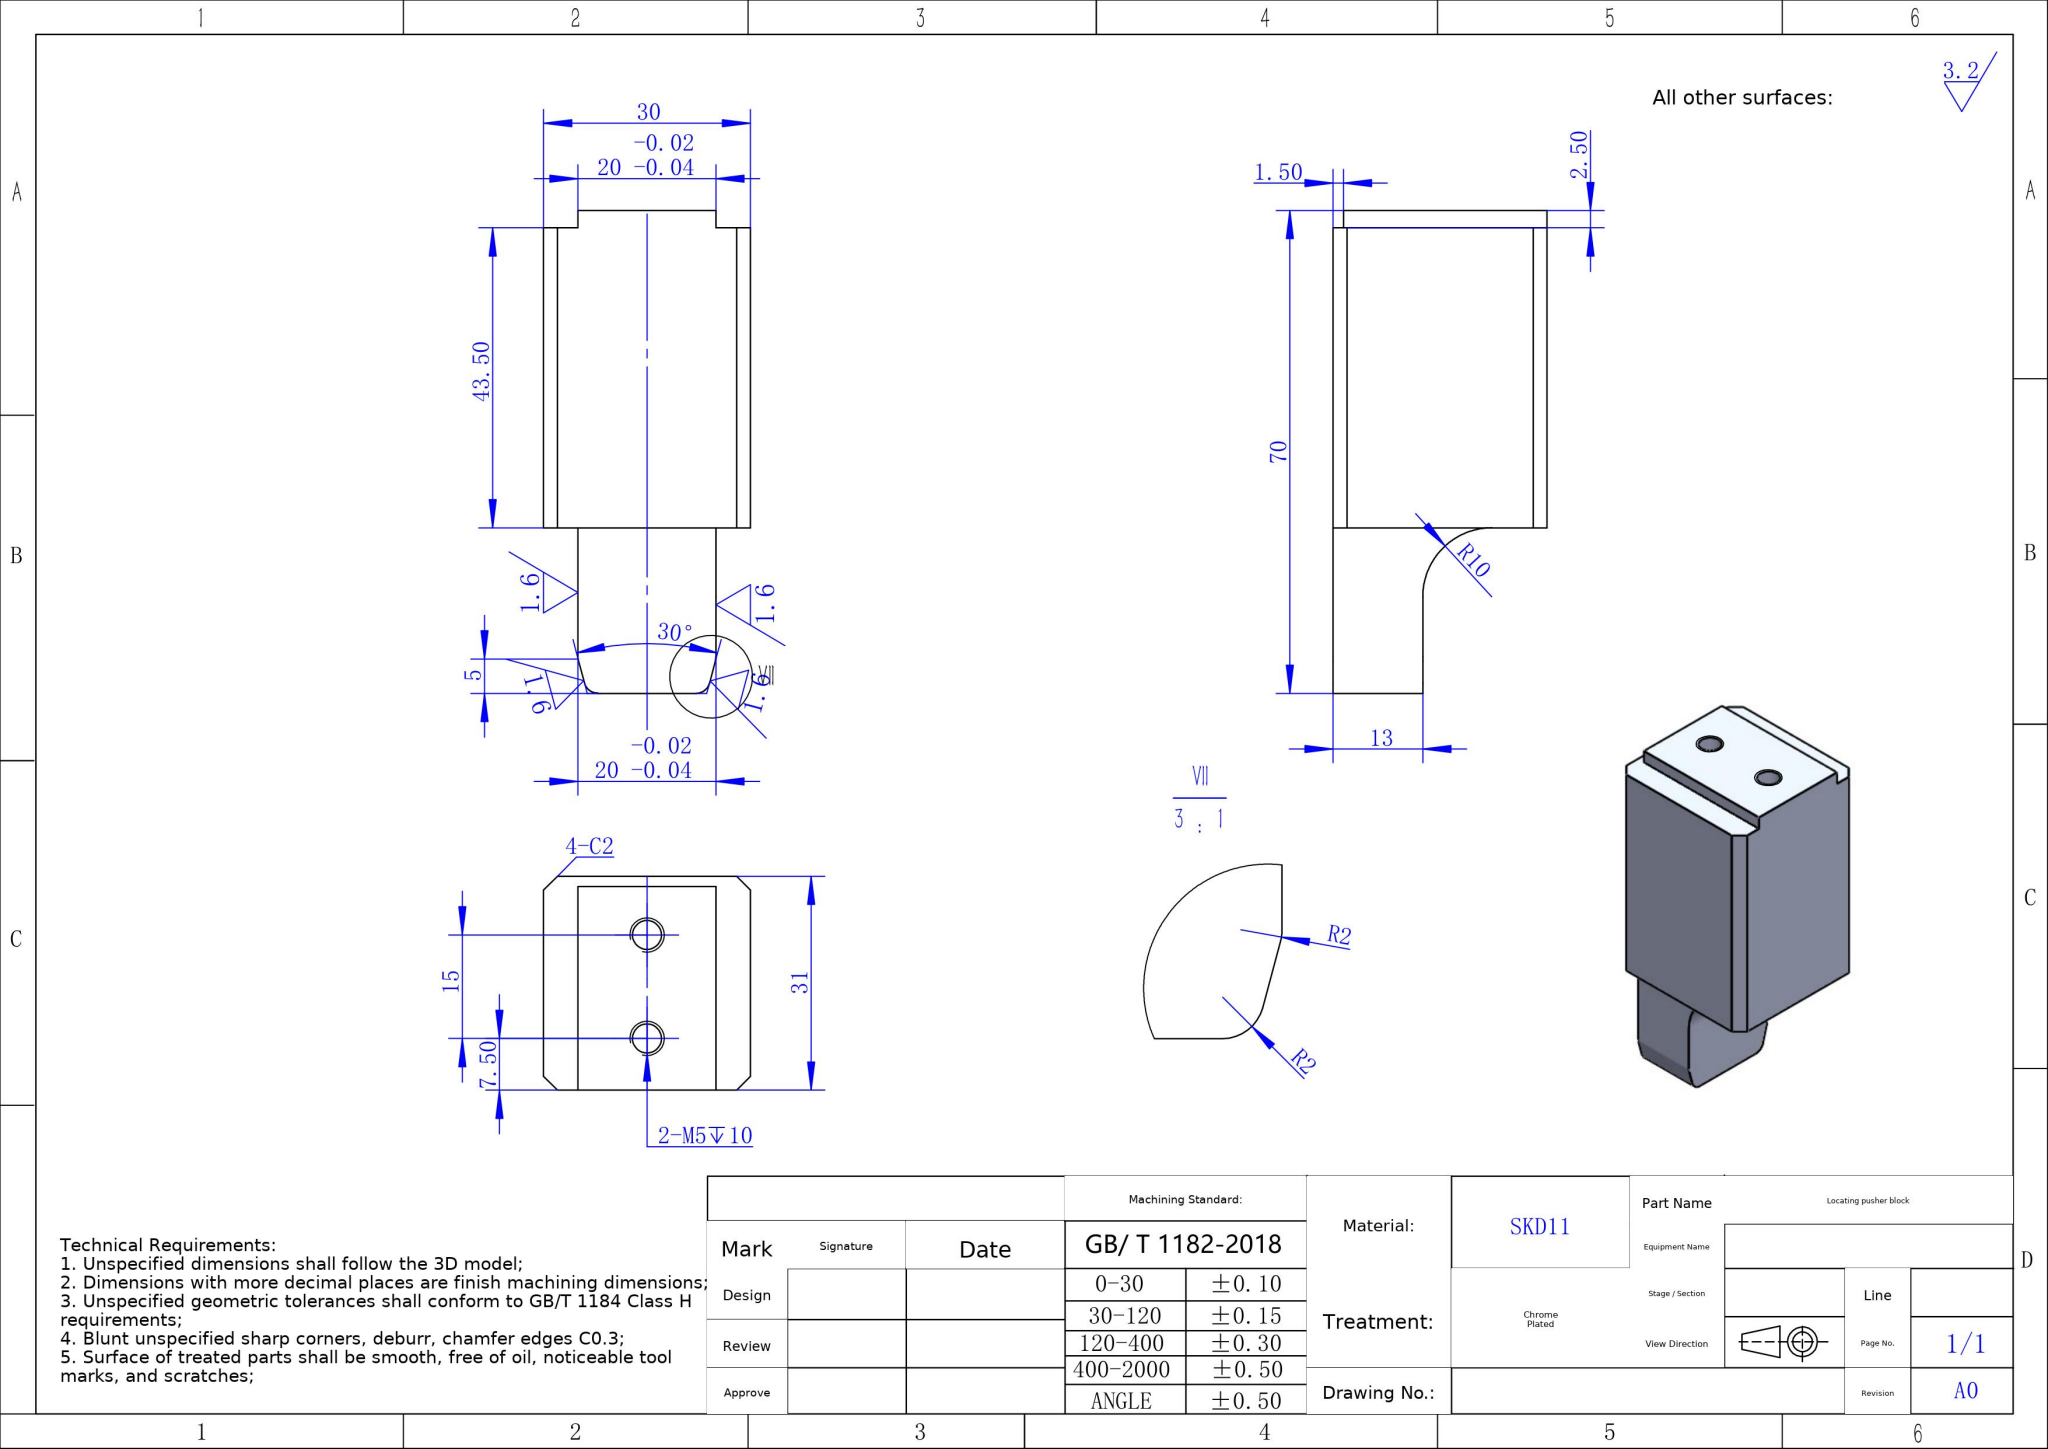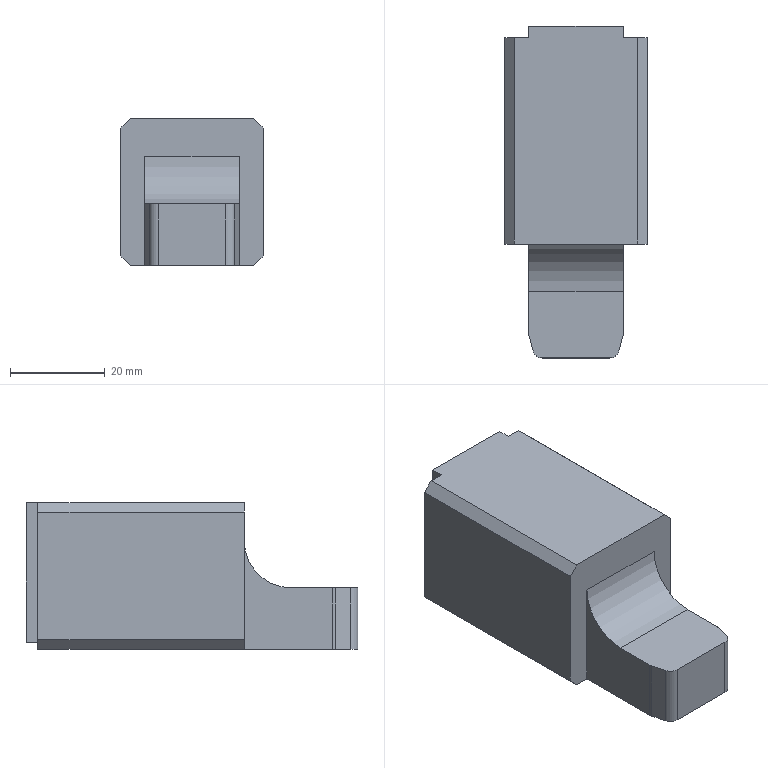Part | SolidWorks | mm | material SKD11 | 1 solid | 33 faces | box 30 x 70 x 31 mm | volume 47753 mm3 | plane 20 | cylinder 9 | cone 4 | commonest cylinder face diameters 4.2 x4 4 x4 20 x1
build123d program:
from build123d import *

# Parameters (mm, degrees)
SKETCH1_W             = 30
SKETCH1_H             = 43.5
BOSS_EXTRUDE1_DEPTH   = 31
CHAMFER1_SIZE         = 2
SKETCH2_W             = 20
SKETCH2_H             = 2.5
BOSS_EXTRUDE2_DEPTH   = 29.5
M5_TAPPED_HOLE1_D     = 4.2
M5_TAPPED_HOLE1_DEPTH = 14
M5_TAPPED_HOLE1_TIP   = 1.262
SKETCH5_W             = 13
SKETCH5_H             = 24
BOSS_EXTRUDE3_DEPTH   = 10
FILLET1_R             = 10
CUT_EXTRUDE1_DEPTH    = 20
FILLET2_R             = 2


with BuildPart() as part:
    # Sketch1 → Boss-Extrude1 (new body)
    with BuildSketch(Plane.XY):
        Rectangle(SKETCH1_W, SKETCH1_H)
    extrude(amount=BOSS_EXTRUDE1_DEPTH)

    # Chamfer1
    chamfer1_edges = [part.edges().sort_by_distance(p)[0] for p in [
        (-15, 0, 31),
        (15, 0, 31),
        (-15, 0, 0),
        (15, 0, 0),
    ]]
    chamfer(chamfer1_edges, length=CHAMFER1_SIZE)

    # Sketch2 → Boss-Extrude2 (add)
    with BuildSketch(Plane.XY.offset(31)):
        with Locations((0, 23)):
            Rectangle(SKETCH2_W, SKETCH2_H)
    extrude(amount=-BOSS_EXTRUDE2_DEPTH)

    # M5 Tapped Hole1
    with Locations(Plane(origin=(0, 24.25, 0), x_dir=(1, 0, 0), z_dir=(0, 1, 0))):
        with Locations((0, -23.5), (0, -8.5)):
            Hole(M5_TAPPED_HOLE1_D / 2, depth=M5_TAPPED_HOLE1_DEPTH)
            with Locations((0, 0, -(M5_TAPPED_HOLE1_DEPTH + M5_TAPPED_HOLE1_TIP / 2))):  # 118° drill point
                Cone(0, M5_TAPPED_HOLE1_D / 2, M5_TAPPED_HOLE1_TIP, mode=Mode.SUBTRACT)

    # Sketch5 → Boss-Extrude3 (add, symmetric)
    with BuildSketch(Plane(origin=(0, 0, 0), x_dir=(0, 0, -1), z_dir=(1, 0, 0))):
        with Locations((-6.5, -33.75)):
            Rectangle(SKETCH5_W, SKETCH5_H)
    extrude(amount=BOSS_EXTRUDE3_DEPTH, both=True)

    # Fillet1
    fillet1_edges = [part.edges().sort_by_distance(p)[0] for p in [
        (0, -21.75, 13),
    ]]
    fillet(fillet1_edges, radius=FILLET1_R)

    # Sketch6 → Cut-Extrude1 (cut)
    with BuildSketch(Plane.XY.offset(13)):
        Polygon((8.66, -45.75), (10, -40.75), (16.367, -43.841), (11.712, -47.429), align=None)
        Polygon((-11.712, -47.429), (-8.66, -45.75), (-10, -40.75), (-16.367, -43.841), align=None)
    extrude(amount=-CUT_EXTRUDE1_DEPTH, mode=Mode.SUBTRACT)

    # Fillet2
    fillet2_edges = [part.edges().sort_by_distance(p)[0] for p in [
        (-8.66, -45.75, 6.5),
        (-10, -40.75, 6.5),
        (10, -40.75, 6.5),
        (8.66, -45.75, 6.5),
    ]]
    fillet(fillet2_edges, radius=FILLET2_R)


solid = part.part
STEP:
#1=CARTESIAN_POINT('',(0.,10.25,21.4));
#2=VERTEX_POINT('',#1);
#3=CARTESIAN_POINT('',(0.,10.25,25.6));
#4=VERTEX_POINT('',#3);
#5=CARTESIAN_POINT('',(0.,10.25,23.5));
#6=DIRECTION('',(0.,1.,0.));
#7=DIRECTION('',(0.,0.,1.));
#8=AXIS2_PLACEMENT_3D('',#5,#6,#7);
#9=CIRCLE('',#8,2.1);
#10=EDGE_CURVE('',#2,#4,#9,.T.);
#11=ORIENTED_EDGE('',*,*,#10,.F.);
#12=CARTESIAN_POINT('',(0.,24.25,21.4));
#13=VERTEX_POINT('',#12);
#14=CARTESIAN_POINT('',(0.,24.25,21.4));
#15=DIRECTION('',(0.,1.,0.));
#16=VECTOR('',#15,1000.);
#17=LINE('',#14,#16);
#18=EDGE_CURVE('',#2,#13,#17,.T.);
#19=ORIENTED_EDGE('',*,*,#18,.T.);
#20=CARTESIAN_POINT('',(0.,24.25,25.6));
#21=VERTEX_POINT('',#20);
#22=CARTESIAN_POINT('',(0.,24.25,23.5));
#23=DIRECTION('',(0.,1.,0.));
#24=DIRECTION('',(0.,0.,1.));
#25=AXIS2_PLACEMENT_3D('',#22,#23,#24);
#26=CIRCLE('',#25,2.1);
#27=EDGE_CURVE('',#13,#21,#26,.T.);
#28=ORIENTED_EDGE('',*,*,#27,.T.);
#29=CARTESIAN_POINT('',(0.,24.25,25.6));
#30=DIRECTION('',(0.,1.,0.));
#31=VECTOR('',#30,1000.);
#32=LINE('',#29,#31);
#33=EDGE_CURVE('',#4,#21,#32,.T.);
#34=ORIENTED_EDGE('',*,*,#33,.F.);
#35=EDGE_LOOP('',(#11,#19,#28,#34));
#36=FACE_OUTER_BOUND('',#35,.T.);
#37=CARTESIAN_POINT('',(0.,24.25,23.5));
#38=DIRECTION('',(0.,1.,0.));
#39=DIRECTION('',(0.,0.,1.));
#40=AXIS2_PLACEMENT_3D('',#37,#38,#39);
#41=CYLINDRICAL_SURFACE('',#40,2.1);
#42=ADVANCED_FACE('',(#36),#41,.F.);
#43=CARTESIAN_POINT('',(-0.,8.988,23.5));
#44=VERTEX_POINT('',#43);
#45=CARTESIAN_POINT('',(0.,10.25,25.6));
#46=DIRECTION('',(0.,0.515,0.8572));
#47=VECTOR('',#46,1000.);
#48=LINE('',#45,#47);
#49=EDGE_CURVE('',#44,#4,#48,.T.);
#50=ORIENTED_EDGE('',*,*,#49,.F.);
#51=CARTESIAN_POINT('',(0.,10.25,21.4));
#52=DIRECTION('',(0.,0.515,-0.8572));
#53=VECTOR('',#52,1000.);
#54=LINE('',#51,#53);
#55=EDGE_CURVE('',#44,#2,#54,.T.);
#56=ORIENTED_EDGE('',*,*,#55,.T.);
#57=ORIENTED_EDGE('',*,*,#10,.T.);
#58=EDGE_LOOP('',(#50,#56,#57));
#59=FACE_OUTER_BOUND('',#58,.T.);
#60=CARTESIAN_POINT('',(0.,10.25,23.5));
#61=DIRECTION('',(0.,1.,0.));
#62=DIRECTION('',(0.,0.,1.));
#63=AXIS2_PLACEMENT_3D('',#60,#61,#62);
#64=CONICAL_SURFACE('',#63,2.1,1.03);
#65=ADVANCED_FACE('',(#59),#64,.F.);
#66=CARTESIAN_POINT('',(0.,10.25,6.4));
#67=VERTEX_POINT('',#66);
#68=CARTESIAN_POINT('',(0.,10.25,10.6));
#69=VERTEX_POINT('',#68);
#70=CARTESIAN_POINT('',(0.,10.25,8.5));
#71=DIRECTION('',(0.,1.,0.));
#72=DIRECTION('',(0.,0.,1.));
#73=AXIS2_PLACEMENT_3D('',#70,#71,#72);
#74=CIRCLE('',#73,2.1);
#75=EDGE_CURVE('',#67,#69,#74,.T.);
#76=ORIENTED_EDGE('',*,*,#75,.F.);
#77=CARTESIAN_POINT('',(0.,24.25,6.4));
#78=VERTEX_POINT('',#77);
#79=CARTESIAN_POINT('',(0.,24.25,6.4));
#80=DIRECTION('',(0.,1.,0.));
#81=VECTOR('',#80,1000.);
#82=LINE('',#79,#81);
#83=EDGE_CURVE('',#67,#78,#82,.T.);
#84=ORIENTED_EDGE('',*,*,#83,.T.);
#85=CARTESIAN_POINT('',(0.,24.25,10.6));
#86=VERTEX_POINT('',#85);
#87=CARTESIAN_POINT('',(0.,24.25,8.5));
#88=DIRECTION('',(0.,1.,0.));
#89=DIRECTION('',(0.,0.,1.));
#90=AXIS2_PLACEMENT_3D('',#87,#88,#89);
#91=CIRCLE('',#90,2.1);
#92=EDGE_CURVE('',#78,#86,#91,.T.);
#93=ORIENTED_EDGE('',*,*,#92,.T.);
#94=CARTESIAN_POINT('',(0.,24.25,10.6));
#95=DIRECTION('',(0.,1.,0.));
#96=VECTOR('',#95,1000.);
#97=LINE('',#94,#96);
#98=EDGE_CURVE('',#69,#86,#97,.T.);
#99=ORIENTED_EDGE('',*,*,#98,.F.);
#100=EDGE_LOOP('',(#76,#84,#93,#99));
#101=FACE_OUTER_BOUND('',#100,.T.);
#102=CARTESIAN_POINT('',(0.,24.25,8.5));
#103=DIRECTION('',(0.,1.,0.));
#104=DIRECTION('',(0.,0.,1.));
#105=AXIS2_PLACEMENT_3D('',#102,#103,#104);
#106=CYLINDRICAL_SURFACE('',#105,2.1);
#107=ADVANCED_FACE('',(#101),#106,.F.);
#108=CARTESIAN_POINT('',(-0.,8.988,8.5));
#109=VERTEX_POINT('',#108);
#110=CARTESIAN_POINT('',(0.,10.25,10.6));
#111=DIRECTION('',(0.,0.515,0.8572));
#112=VECTOR('',#111,1000.);
#113=LINE('',#110,#112);
#114=EDGE_CURVE('',#109,#69,#113,.T.);
#115=ORIENTED_EDGE('',*,*,#114,.F.);
#116=CARTESIAN_POINT('',(0.,10.25,6.4));
#117=DIRECTION('',(0.,0.515,-0.8572));
#118=VECTOR('',#117,1000.);
#119=LINE('',#116,#118);
#120=EDGE_CURVE('',#109,#67,#119,.T.);
#121=ORIENTED_EDGE('',*,*,#120,.T.);
#122=ORIENTED_EDGE('',*,*,#75,.T.);
#123=EDGE_LOOP('',(#115,#121,#122));
#124=FACE_OUTER_BOUND('',#123,.T.);
#125=CARTESIAN_POINT('',(0.,10.25,8.5));
#126=DIRECTION('',(0.,1.,0.));
#127=DIRECTION('',(0.,0.,1.));
#128=AXIS2_PLACEMENT_3D('',#125,#126,#127);
#129=CONICAL_SURFACE('',#128,2.1,1.03);
#130=ADVANCED_FACE('',(#124),#129,.F.);
#131=CARTESIAN_POINT('',(-10.,21.75,1.5));
#132=VERTEX_POINT('',#131);
#133=CARTESIAN_POINT('',(-10.,21.75,31.));
#134=VERTEX_POINT('',#133);
#135=CARTESIAN_POINT('',(-10.,21.75,1.5));
#136=DIRECTION('',(0.,0.,1.));
#137=VECTOR('',#136,1000.);
#138=LINE('',#135,#137);
#139=EDGE_CURVE('',#132,#134,#138,.T.);
#140=ORIENTED_EDGE('',*,*,#139,.F.);
#141=CARTESIAN_POINT('',(10.,21.75,1.5));
#142=VERTEX_POINT('',#141);
#143=CARTESIAN_POINT('',(-10.,21.75,1.5));
#144=DIRECTION('',(1.,0.,0.));
#145=VECTOR('',#144,1000.);
#146=LINE('',#143,#145);
#147=EDGE_CURVE('',#132,#142,#146,.T.);
#148=ORIENTED_EDGE('',*,*,#147,.T.);
#149=CARTESIAN_POINT('',(10.,21.75,31.));
#150=VERTEX_POINT('',#149);
#151=CARTESIAN_POINT('',(10.,21.75,1.5));
#152=DIRECTION('',(0.,0.,1.));
#153=VECTOR('',#152,1000.);
#154=LINE('',#151,#153);
#155=EDGE_CURVE('',#142,#150,#154,.T.);
#156=ORIENTED_EDGE('',*,*,#155,.T.);
#157=CARTESIAN_POINT('',(13.,21.75,31.));
#158=VERTEX_POINT('',#157);
#159=CARTESIAN_POINT('',(-15.,21.75,31.));
#160=DIRECTION('',(-1.,0.,0.));
#161=VECTOR('',#160,1000.);
#162=LINE('',#159,#161);
#163=EDGE_CURVE('',#158,#150,#162,.T.);
#164=ORIENTED_EDGE('',*,*,#163,.F.);
#165=CARTESIAN_POINT('',(15.,21.75,29.));
#166=VERTEX_POINT('',#165);
#167=CARTESIAN_POINT('',(13.,21.75,31.));
#168=DIRECTION('',(0.7071,0.,-0.7071));
#169=VECTOR('',#168,1000.);
#170=LINE('',#167,#169);
#171=EDGE_CURVE('',#158,#166,#170,.T.);
#172=ORIENTED_EDGE('',*,*,#171,.T.);
#173=CARTESIAN_POINT('',(15.,21.75,2.));
#174=VERTEX_POINT('',#173);
#175=CARTESIAN_POINT('',(15.,21.75,31.));
#176=DIRECTION('',(0.,0.,-1.));
#177=VECTOR('',#176,1000.);
#178=LINE('',#175,#177);
#179=EDGE_CURVE('',#166,#174,#178,.T.);
#180=ORIENTED_EDGE('',*,*,#179,.T.);
#181=CARTESIAN_POINT('',(13.,21.75,0.));
#182=VERTEX_POINT('',#181);
#183=CARTESIAN_POINT('',(15.,21.75,2.));
#184=DIRECTION('',(-0.7071,0.,-0.7071));
#185=VECTOR('',#184,1000.);
#186=LINE('',#183,#185);
#187=EDGE_CURVE('',#174,#182,#186,.T.);
#188=ORIENTED_EDGE('',*,*,#187,.T.);
#189=CARTESIAN_POINT('',(-13.,21.75,0.));
#190=VERTEX_POINT('',#189);
#191=CARTESIAN_POINT('',(-15.,21.75,0.));
#192=DIRECTION('',(-1.,0.,0.));
#193=VECTOR('',#192,1000.);
#194=LINE('',#191,#193);
#195=EDGE_CURVE('',#182,#190,#194,.T.);
#196=ORIENTED_EDGE('',*,*,#195,.T.);
#197=CARTESIAN_POINT('',(-15.,21.75,2.));
#198=VERTEX_POINT('',#197);
#199=CARTESIAN_POINT('',(-15.,21.75,2.));
#200=DIRECTION('',(-0.7071,0.,0.7071));
#201=VECTOR('',#200,1000.);
#202=LINE('',#199,#201);
#203=EDGE_CURVE('',#190,#198,#202,.T.);
#204=ORIENTED_EDGE('',*,*,#203,.T.);
#205=CARTESIAN_POINT('',(-15.,21.75,29.));
#206=VERTEX_POINT('',#205);
#207=CARTESIAN_POINT('',(-15.,21.75,31.));
#208=DIRECTION('',(0.,0.,-1.));
#209=VECTOR('',#208,1000.);
#210=LINE('',#207,#209);
#211=EDGE_CURVE('',#206,#198,#210,.T.);
#212=ORIENTED_EDGE('',*,*,#211,.F.);
#213=CARTESIAN_POINT('',(-13.,21.75,31.));
#214=VERTEX_POINT('',#213);
#215=CARTESIAN_POINT('',(-13.,21.75,31.));
#216=DIRECTION('',(0.7071,0.,0.7071));
#217=VECTOR('',#216,1000.);
#218=LINE('',#215,#217);
#219=EDGE_CURVE('',#206,#214,#218,.T.);
#220=ORIENTED_EDGE('',*,*,#219,.T.);
#221=CARTESIAN_POINT('',(-15.,21.75,31.));
#222=DIRECTION('',(-1.,0.,0.));
#223=VECTOR('',#222,1000.);
#224=LINE('',#221,#223);
#225=EDGE_CURVE('',#134,#214,#224,.T.);
#226=ORIENTED_EDGE('',*,*,#225,.F.);
#227=EDGE_LOOP('',(#140,#148,#156,#164,#172,#180,#188,#196,#204,#212,#220,#226));
#228=FACE_OUTER_BOUND('',#227,.T.);
#229=CARTESIAN_POINT('',(-15.,21.75,31.));
#230=DIRECTION('',(0.,-1.,0.));
#231=DIRECTION('',(0.,0.,-1.));
#232=AXIS2_PLACEMENT_3D('',#229,#230,#231);
#233=PLANE('',#232);
#234=ADVANCED_FACE('',(#228),#233,.F.);
#235=CARTESIAN_POINT('',(15.,-21.75,29.));
#236=VERTEX_POINT('',#235);
#237=CARTESIAN_POINT('',(15.,-21.75,2.));
#238=VERTEX_POINT('',#237);
#239=CARTESIAN_POINT('',(15.,-21.75,31.));
#240=DIRECTION('',(0.,0.,-1.));
#241=VECTOR('',#240,1000.);
#242=LINE('',#239,#241);
#243=EDGE_CURVE('',#236,#238,#242,.T.);
#244=ORIENTED_EDGE('',*,*,#243,.T.);
#245=CARTESIAN_POINT('',(15.,21.75,2.));
#246=DIRECTION('',(-0.,1.,0.));
#247=VECTOR('',#246,1000.);
#248=LINE('',#245,#247);
#249=EDGE_CURVE('',#238,#174,#248,.T.);
#250=ORIENTED_EDGE('',*,*,#249,.T.);
#251=ORIENTED_EDGE('',*,*,#179,.F.);
#252=CARTESIAN_POINT('',(15.,-21.75,29.));
#253=DIRECTION('',(0.,-1.,0.));
#254=VECTOR('',#253,1000.);
#255=LINE('',#252,#254);
#256=EDGE_CURVE('',#166,#236,#255,.T.);
#257=ORIENTED_EDGE('',*,*,#256,.T.);
#258=EDGE_LOOP('',(#244,#250,#251,#257));
#259=FACE_OUTER_BOUND('',#258,.T.);
#260=CARTESIAN_POINT('',(15.,21.75,31.));
#261=DIRECTION('',(-1.,-0.,0.));
#262=DIRECTION('',(0.,-1.,0.));
#263=AXIS2_PLACEMENT_3D('',#260,#261,#262);
#264=PLANE('',#263);
#265=ADVANCED_FACE('',(#259),#264,.F.);
#266=ORIENTED_EDGE('',*,*,#211,.T.);
#267=CARTESIAN_POINT('',(-15.,-21.75,2.));
#268=VERTEX_POINT('',#267);
#269=CARTESIAN_POINT('',(-15.,21.75,2.));
#270=DIRECTION('',(0.,-1.,0.));
#271=VECTOR('',#270,1000.);
#272=LINE('',#269,#271);
#273=EDGE_CURVE('',#198,#268,#272,.T.);
#274=ORIENTED_EDGE('',*,*,#273,.T.);
#275=CARTESIAN_POINT('',(-15.,-21.75,29.));
#276=VERTEX_POINT('',#275);
#277=CARTESIAN_POINT('',(-15.,-21.75,31.));
#278=DIRECTION('',(0.,0.,-1.));
#279=VECTOR('',#278,1000.);
#280=LINE('',#277,#279);
#281=EDGE_CURVE('',#276,#268,#280,.T.);
#282=ORIENTED_EDGE('',*,*,#281,.F.);
#283=CARTESIAN_POINT('',(-15.,21.75,29.));
#284=DIRECTION('',(-0.,1.,0.));
#285=VECTOR('',#284,1000.);
#286=LINE('',#283,#285);
#287=EDGE_CURVE('',#276,#206,#286,.T.);
#288=ORIENTED_EDGE('',*,*,#287,.T.);
#289=EDGE_LOOP('',(#266,#274,#282,#288));
#290=FACE_OUTER_BOUND('',#289,.T.);
#291=CARTESIAN_POINT('',(-15.,21.75,31.));
#292=DIRECTION('',(1.,0.,0.));
#293=DIRECTION('',(-0.,1.,0.));
#294=AXIS2_PLACEMENT_3D('',#291,#292,#293);
#295=PLANE('',#294);
#296=ADVANCED_FACE('',(#290),#295,.F.);
#297=CARTESIAN_POINT('',(-10.,-21.75,0.));
#298=VERTEX_POINT('',#297);
#299=CARTESIAN_POINT('',(-10.,-21.75,23.));
#300=VERTEX_POINT('',#299);
#301=CARTESIAN_POINT('',(-10.,-21.75,13.));
#302=DIRECTION('',(0.,0.,1.));
#303=VECTOR('',#302,1000.);
#304=LINE('',#301,#303);
#305=EDGE_CURVE('',#298,#300,#304,.T.);
#306=ORIENTED_EDGE('',*,*,#305,.T.);
#307=CARTESIAN_POINT('',(10.,-21.75,23.));
#308=VERTEX_POINT('',#307);
#309=CARTESIAN_POINT('',(10.,-21.75,23.));
#310=DIRECTION('',(1.,0.,0.));
#311=VECTOR('',#310,1000.);
#312=LINE('',#309,#311);
#313=EDGE_CURVE('',#300,#308,#312,.T.);
#314=ORIENTED_EDGE('',*,*,#313,.T.);
#315=CARTESIAN_POINT('',(10.,-21.75,0.));
#316=VERTEX_POINT('',#315);
#317=CARTESIAN_POINT('',(10.,-21.75,13.));
#318=DIRECTION('',(0.,0.,1.));
#319=VECTOR('',#318,1000.);
#320=LINE('',#317,#319);
#321=EDGE_CURVE('',#316,#308,#320,.T.);
#322=ORIENTED_EDGE('',*,*,#321,.F.);
#323=CARTESIAN_POINT('',(13.,-21.75,0.));
#324=VERTEX_POINT('',#323);
#325=CARTESIAN_POINT('',(-15.,-21.75,0.));
#326=DIRECTION('',(1.,0.,0.));
#327=VECTOR('',#326,1000.);
#328=LINE('',#325,#327);
#329=EDGE_CURVE('',#316,#324,#328,.T.);
#330=ORIENTED_EDGE('',*,*,#329,.T.);
#331=CARTESIAN_POINT('',(15.,-21.75,2.));
#332=DIRECTION('',(0.7071,0.,0.7071));
#333=VECTOR('',#332,1000.);
#334=LINE('',#331,#333);
#335=EDGE_CURVE('',#324,#238,#334,.T.);
#336=ORIENTED_EDGE('',*,*,#335,.T.);
#337=ORIENTED_EDGE('',*,*,#243,.F.);
#338=CARTESIAN_POINT('',(13.,-21.75,31.));
#339=VERTEX_POINT('',#338);
#340=CARTESIAN_POINT('',(13.,-21.75,31.));
#341=DIRECTION('',(-0.7071,0.,0.7071));
#342=VECTOR('',#341,1000.);
#343=LINE('',#340,#342);
#344=EDGE_CURVE('',#236,#339,#343,.T.);
#345=ORIENTED_EDGE('',*,*,#344,.T.);
#346=CARTESIAN_POINT('',(-13.,-21.75,31.));
#347=VERTEX_POINT('',#346);
#348=CARTESIAN_POINT('',(-15.,-21.75,31.));
#349=DIRECTION('',(1.,0.,0.));
#350=VECTOR('',#349,1000.);
#351=LINE('',#348,#350);
#352=EDGE_CURVE('',#347,#339,#351,.T.);
#353=ORIENTED_EDGE('',*,*,#352,.F.);
#354=CARTESIAN_POINT('',(-13.,-21.75,31.));
#355=DIRECTION('',(-0.7071,0.,-0.7071));
#356=VECTOR('',#355,1000.);
#357=LINE('',#354,#356);
#358=EDGE_CURVE('',#347,#276,#357,.T.);
#359=ORIENTED_EDGE('',*,*,#358,.T.);
#360=ORIENTED_EDGE('',*,*,#281,.T.);
#361=CARTESIAN_POINT('',(-13.,-21.75,0.));
#362=VERTEX_POINT('',#361);
#363=CARTESIAN_POINT('',(-15.,-21.75,2.));
#364=DIRECTION('',(0.7071,0.,-0.7071));
#365=VECTOR('',#364,1000.);
#366=LINE('',#363,#365);
#367=EDGE_CURVE('',#268,#362,#366,.T.);
#368=ORIENTED_EDGE('',*,*,#367,.T.);
#369=CARTESIAN_POINT('',(-15.,-21.75,0.));
#370=DIRECTION('',(1.,0.,0.));
#371=VECTOR('',#370,1000.);
#372=LINE('',#369,#371);
#373=EDGE_CURVE('',#362,#298,#372,.T.);
#374=ORIENTED_EDGE('',*,*,#373,.T.);
#375=EDGE_LOOP('',(#306,#314,#322,#330,#336,#337,#345,#353,#359,#360,#368,#374));
#376=FACE_OUTER_BOUND('',#375,.T.);
#377=CARTESIAN_POINT('',(-15.,-21.75,31.));
#378=DIRECTION('',(0.,1.,0.));
#379=DIRECTION('',(0.,0.,1.));
#380=AXIS2_PLACEMENT_3D('',#377,#378,#379);
#381=PLANE('',#380);
#382=ADVANCED_FACE('',(#376),#381,.F.);
#383=ORIENTED_EDGE('',*,*,#352,.T.);
#384=CARTESIAN_POINT('',(13.,21.75,31.));
#385=DIRECTION('',(-0.,1.,0.));
#386=VECTOR('',#385,1000.);
#387=LINE('',#384,#386);
#388=EDGE_CURVE('',#339,#158,#387,.T.);
#389=ORIENTED_EDGE('',*,*,#388,.T.);
#390=ORIENTED_EDGE('',*,*,#163,.T.);
#391=CARTESIAN_POINT('',(10.,24.25,31.));
#392=VERTEX_POINT('',#391);
#393=CARTESIAN_POINT('',(10.,24.25,31.));
#394=DIRECTION('',(-0.,1.,0.));
#395=VECTOR('',#394,1000.);
#396=LINE('',#393,#395);
#397=EDGE_CURVE('',#150,#392,#396,.T.);
#398=ORIENTED_EDGE('',*,*,#397,.T.);
#399=CARTESIAN_POINT('',(-10.,24.25,31.));
#400=VERTEX_POINT('',#399);
#401=CARTESIAN_POINT('',(-10.,24.25,31.));
#402=DIRECTION('',(-1.,0.,0.));
#403=VECTOR('',#402,1000.);
#404=LINE('',#401,#403);
#405=EDGE_CURVE('',#392,#400,#404,.T.);
#406=ORIENTED_EDGE('',*,*,#405,.T.);
#407=CARTESIAN_POINT('',(-10.,24.25,31.));
#408=DIRECTION('',(0.,-1.,0.));
#409=VECTOR('',#408,1000.);
#410=LINE('',#407,#409);
#411=EDGE_CURVE('',#400,#134,#410,.T.);
#412=ORIENTED_EDGE('',*,*,#411,.T.);
#413=ORIENTED_EDGE('',*,*,#225,.T.);
#414=CARTESIAN_POINT('',(-13.,-21.75,31.));
#415=DIRECTION('',(0.,-1.,0.));
#416=VECTOR('',#415,1000.);
#417=LINE('',#414,#416);
#418=EDGE_CURVE('',#214,#347,#417,.T.);
#419=ORIENTED_EDGE('',*,*,#418,.T.);
#420=EDGE_LOOP('',(#383,#389,#390,#398,#406,#412,#413,#419));
#421=FACE_OUTER_BOUND('',#420,.T.);
#422=CARTESIAN_POINT('',(0.,0.,31.));
#423=DIRECTION('',(0.,0.,1.));
#424=DIRECTION('',(1.,0.,0.));
#425=AXIS2_PLACEMENT_3D('',#422,#423,#424);
#426=PLANE('',#425);
#427=ADVANCED_FACE('',(#421),#426,.T.);
#428=CARTESIAN_POINT('',(7.126,-45.75,-0.));
#429=VERTEX_POINT('',#428);
#430=CARTESIAN_POINT('',(-7.126,-45.75,-0.));
#431=VERTEX_POINT('',#430);
#432=CARTESIAN_POINT('',(10.,-45.75,-0.));
#433=DIRECTION('',(-1.,0.,0.));
#434=VECTOR('',#433,1000.);
#435=LINE('',#432,#434);
#436=EDGE_CURVE('',#429,#431,#435,.T.);
#437=ORIENTED_EDGE('',*,*,#436,.T.);
#438=CARTESIAN_POINT('',(-9.057,-44.268,0.));
#439=VERTEX_POINT('',#438);
#440=CARTESIAN_POINT('',(-7.126,-43.75,0.));
#441=DIRECTION('',(0.,0.,-1.));
#442=DIRECTION('',(1.,0.,0.));
#443=AXIS2_PLACEMENT_3D('',#440,#441,#442);
#444=CIRCLE('',#443,2.);
#445=EDGE_CURVE('',#431,#439,#444,.T.);
#446=ORIENTED_EDGE('',*,*,#445,.T.);
#447=CARTESIAN_POINT('',(-9.932,-41.004,0.));
#448=VERTEX_POINT('',#447);
#449=CARTESIAN_POINT('',(-19.518,-5.23,0.));
#450=DIRECTION('',(-0.2588,0.9659,0.));
#451=VECTOR('',#450,1000.);
#452=LINE('',#449,#451);
#453=EDGE_CURVE('',#439,#448,#452,.T.);
#454=ORIENTED_EDGE('',*,*,#453,.T.);
#455=CARTESIAN_POINT('',(-10.,-40.487,-0.));
#456=VERTEX_POINT('',#455);
#457=CARTESIAN_POINT('',(-8.,-40.487,0.));
#458=DIRECTION('',(0.,0.,-1.));
#459=DIRECTION('',(1.,0.,0.));
#460=AXIS2_PLACEMENT_3D('',#457,#458,#459);
#461=CIRCLE('',#460,2.);
#462=EDGE_CURVE('',#448,#456,#461,.T.);
#463=ORIENTED_EDGE('',*,*,#462,.T.);
#464=CARTESIAN_POINT('',(-10.,-21.75,0.));
#465=DIRECTION('',(0.,1.,0.));
#466=VECTOR('',#465,1000.);
#467=LINE('',#464,#466);
#468=EDGE_CURVE('',#456,#298,#467,.T.);
#469=ORIENTED_EDGE('',*,*,#468,.T.);
#470=ORIENTED_EDGE('',*,*,#373,.F.);
#471=CARTESIAN_POINT('',(-13.,-0.,0.));
#472=DIRECTION('',(-0.,1.,0.));
#473=VECTOR('',#472,1000.);
#474=LINE('',#471,#473);
#475=EDGE_CURVE('',#362,#190,#474,.T.);
#476=ORIENTED_EDGE('',*,*,#475,.T.);
#477=ORIENTED_EDGE('',*,*,#195,.F.);
#478=CARTESIAN_POINT('',(13.,0.,0.));
#479=DIRECTION('',(0.,-1.,0.));
#480=VECTOR('',#479,1000.);
#481=LINE('',#478,#480);
#482=EDGE_CURVE('',#182,#324,#481,.T.);
#483=ORIENTED_EDGE('',*,*,#482,.T.);
#484=ORIENTED_EDGE('',*,*,#329,.F.);
#485=CARTESIAN_POINT('',(10.,-40.487,-0.));
#486=VERTEX_POINT('',#485);
#487=CARTESIAN_POINT('',(10.,-21.75,0.));
#488=DIRECTION('',(0.,1.,0.));
#489=VECTOR('',#488,1000.);
#490=LINE('',#487,#489);
#491=EDGE_CURVE('',#486,#316,#490,.T.);
#492=ORIENTED_EDGE('',*,*,#491,.F.);
#493=CARTESIAN_POINT('',(9.932,-41.004,0.));
#494=VERTEX_POINT('',#493);
#495=CARTESIAN_POINT('',(8.,-40.487,0.));
#496=DIRECTION('',(0.,0.,-1.));
#497=DIRECTION('',(1.,0.,0.));
#498=AXIS2_PLACEMENT_3D('',#495,#496,#497);
#499=CIRCLE('',#498,2.);
#500=EDGE_CURVE('',#486,#494,#499,.T.);
#501=ORIENTED_EDGE('',*,*,#500,.T.);
#502=CARTESIAN_POINT('',(9.057,-44.268,0.));
#503=VERTEX_POINT('',#502);
#504=CARTESIAN_POINT('',(19.518,-5.23,0.));
#505=DIRECTION('',(-0.2588,-0.9659,0.));
#506=VECTOR('',#505,1000.);
#507=LINE('',#504,#506);
#508=EDGE_CURVE('',#494,#503,#507,.T.);
#509=ORIENTED_EDGE('',*,*,#508,.T.);
#510=CARTESIAN_POINT('',(7.126,-43.75,0.));
#511=DIRECTION('',(0.,0.,-1.));
#512=DIRECTION('',(1.,0.,0.));
#513=AXIS2_PLACEMENT_3D('',#510,#511,#512);
#514=CIRCLE('',#513,2.);
#515=EDGE_CURVE('',#503,#429,#514,.T.);
#516=ORIENTED_EDGE('',*,*,#515,.T.);
#517=EDGE_LOOP('',(#437,#446,#454,#463,#469,#470,#476,#477,#483,#484,#492,#501,#509,#516));
#518=FACE_OUTER_BOUND('',#517,.T.);
#519=CARTESIAN_POINT('',(0.,0.,0.));
#520=DIRECTION('',(0.,0.,1.));
#521=DIRECTION('',(1.,0.,0.));
#522=AXIS2_PLACEMENT_3D('',#519,#520,#521);
#523=PLANE('',#522);
#524=ADVANCED_FACE('',(#518),#523,.F.);
#525=ORIENTED_EDGE('',*,*,#335,.F.);
#526=ORIENTED_EDGE('',*,*,#482,.F.);
#527=ORIENTED_EDGE('',*,*,#187,.F.);
#528=ORIENTED_EDGE('',*,*,#249,.F.);
#529=EDGE_LOOP('',(#525,#526,#527,#528));
#530=FACE_OUTER_BOUND('',#529,.T.);
#531=CARTESIAN_POINT('',(15.,21.75,2.));
#532=DIRECTION('',(-0.7071,-0.,0.7071));
#533=DIRECTION('',(-0.,1.,0.));
#534=AXIS2_PLACEMENT_3D('',#531,#532,#533);
#535=PLANE('',#534);
#536=ADVANCED_FACE('',(#530),#535,.F.);
#537=ORIENTED_EDGE('',*,*,#344,.F.);
#538=ORIENTED_EDGE('',*,*,#256,.F.);
#539=ORIENTED_EDGE('',*,*,#171,.F.);
#540=ORIENTED_EDGE('',*,*,#388,.F.);
#541=EDGE_LOOP('',(#537,#538,#539,#540));
#542=FACE_OUTER_BOUND('',#541,.T.);
#543=CARTESIAN_POINT('',(13.,0.,31.));
#544=DIRECTION('',(0.7071,0.,0.7071));
#545=DIRECTION('',(0.,-1.,0.));
#546=AXIS2_PLACEMENT_3D('',#543,#544,#545);
#547=PLANE('',#546);
#548=ADVANCED_FACE('',(#542),#547,.T.);
#549=ORIENTED_EDGE('',*,*,#203,.F.);
#550=ORIENTED_EDGE('',*,*,#475,.F.);
#551=ORIENTED_EDGE('',*,*,#367,.F.);
#552=ORIENTED_EDGE('',*,*,#273,.F.);
#553=EDGE_LOOP('',(#549,#550,#551,#552));
#554=FACE_OUTER_BOUND('',#553,.T.);
#555=CARTESIAN_POINT('',(-15.,21.75,2.));
#556=DIRECTION('',(0.7071,0.,0.7071));
#557=DIRECTION('',(0.,-1.,0.));
#558=AXIS2_PLACEMENT_3D('',#555,#556,#557);
#559=PLANE('',#558);
#560=ADVANCED_FACE('',(#554),#559,.F.);
#561=ORIENTED_EDGE('',*,*,#219,.F.);
#562=ORIENTED_EDGE('',*,*,#287,.F.);
#563=ORIENTED_EDGE('',*,*,#358,.F.);
#564=ORIENTED_EDGE('',*,*,#418,.F.);
#565=EDGE_LOOP('',(#561,#562,#563,#564));
#566=FACE_OUTER_BOUND('',#565,.T.);
#567=CARTESIAN_POINT('',(-13.,-0.,31.));
#568=DIRECTION('',(-0.7071,-0.,0.7071));
#569=DIRECTION('',(-0.,1.,0.));
#570=AXIS2_PLACEMENT_3D('',#567,#568,#569);
#571=PLANE('',#570);
#572=ADVANCED_FACE('',(#566),#571,.T.);
#573=ORIENTED_EDGE('',*,*,#397,.F.);
#574=ORIENTED_EDGE('',*,*,#155,.F.);
#575=CARTESIAN_POINT('',(10.,24.25,1.5));
#576=VERTEX_POINT('',#575);
#577=CARTESIAN_POINT('',(10.,24.25,1.5));
#578=DIRECTION('',(-0.,1.,0.));
#579=VECTOR('',#578,1000.);
#580=LINE('',#577,#579);
#581=EDGE_CURVE('',#142,#576,#580,.T.);
#582=ORIENTED_EDGE('',*,*,#581,.T.);
#583=CARTESIAN_POINT('',(10.,24.25,1.5));
#584=DIRECTION('',(0.,0.,1.));
#585=VECTOR('',#584,1000.);
#586=LINE('',#583,#585);
#587=EDGE_CURVE('',#576,#392,#586,.T.);
#588=ORIENTED_EDGE('',*,*,#587,.T.);
#589=EDGE_LOOP('',(#573,#574,#582,#588));
#590=FACE_OUTER_BOUND('',#589,.T.);
#591=CARTESIAN_POINT('',(10.,24.25,1.5));
#592=DIRECTION('',(1.,0.,0.));
#593=DIRECTION('',(-0.,1.,0.));
#594=AXIS2_PLACEMENT_3D('',#591,#592,#593);
#595=PLANE('',#594);
#596=ADVANCED_FACE('',(#590),#595,.T.);
#597=ORIENTED_EDGE('',*,*,#411,.F.);
#598=CARTESIAN_POINT('',(-10.,24.25,1.5));
#599=VERTEX_POINT('',#598);
#600=CARTESIAN_POINT('',(-10.,24.25,1.5));
#601=DIRECTION('',(0.,0.,1.));
#602=VECTOR('',#601,1000.);
#603=LINE('',#600,#602);
#604=EDGE_CURVE('',#599,#400,#603,.T.);
#605=ORIENTED_EDGE('',*,*,#604,.F.);
#606=CARTESIAN_POINT('',(-10.,24.25,1.5));
#607=DIRECTION('',(0.,-1.,0.));
#608=VECTOR('',#607,1000.);
#609=LINE('',#606,#608);
#610=EDGE_CURVE('',#599,#132,#609,.T.);
#611=ORIENTED_EDGE('',*,*,#610,.T.);
#612=ORIENTED_EDGE('',*,*,#139,.T.);
#613=EDGE_LOOP('',(#597,#605,#611,#612));
#614=FACE_OUTER_BOUND('',#613,.T.);
#615=CARTESIAN_POINT('',(-10.,24.25,1.5));
#616=DIRECTION('',(-1.,0.,0.));
#617=DIRECTION('',(0.,0.,1.));
#618=AXIS2_PLACEMENT_3D('',#615,#616,#617);
#619=PLANE('',#618);
#620=ADVANCED_FACE('',(#614),#619,.T.);
#621=CARTESIAN_POINT('',(0.,24.25,23.5));
#622=DIRECTION('',(0.,1.,0.));
#623=DIRECTION('',(0.,0.,1.));
#624=AXIS2_PLACEMENT_3D('',#621,#622,#623);
#625=CIRCLE('',#624,2.1);
#626=EDGE_CURVE('',#21,#13,#625,.T.);
#627=ORIENTED_EDGE('',*,*,#626,.F.);
#628=ORIENTED_EDGE('',*,*,#27,.F.);
#629=EDGE_LOOP('',(#627,#628));
#630=FACE_BOUND('',#629,.T.);
#631=CARTESIAN_POINT('',(0.,24.25,8.5));
#632=DIRECTION('',(0.,1.,0.));
#633=DIRECTION('',(0.,0.,1.));
#634=AXIS2_PLACEMENT_3D('',#631,#632,#633);
#635=CIRCLE('',#634,2.1);
#636=EDGE_CURVE('',#86,#78,#635,.T.);
#637=ORIENTED_EDGE('',*,*,#636,.F.);
#638=ORIENTED_EDGE('',*,*,#92,.F.);
#639=EDGE_LOOP('',(#637,#638));
#640=FACE_BOUND('',#639,.T.);
#641=ORIENTED_EDGE('',*,*,#405,.F.);
#642=ORIENTED_EDGE('',*,*,#587,.F.);
#643=CARTESIAN_POINT('',(-10.,24.25,1.5));
#644=DIRECTION('',(-1.,0.,0.));
#645=VECTOR('',#644,1000.);
#646=LINE('',#643,#645);
#647=EDGE_CURVE('',#576,#599,#646,.T.);
#648=ORIENTED_EDGE('',*,*,#647,.T.);
#649=ORIENTED_EDGE('',*,*,#604,.T.);
#650=EDGE_LOOP('',(#641,#642,#648,#649));
#651=FACE_OUTER_BOUND('',#650,.T.);
#652=CARTESIAN_POINT('',(-10.,24.25,1.5));
#653=DIRECTION('',(0.,1.,0.));
#654=DIRECTION('',(0.,0.,1.));
#655=AXIS2_PLACEMENT_3D('',#652,#653,#654);
#656=PLANE('',#655);
#657=ADVANCED_FACE('',(#630,#640,#651),#656,.T.);
#658=ORIENTED_EDGE('',*,*,#581,.F.);
#659=ORIENTED_EDGE('',*,*,#147,.F.);
#660=ORIENTED_EDGE('',*,*,#610,.F.);
#661=ORIENTED_EDGE('',*,*,#647,.F.);
#662=EDGE_LOOP('',(#658,#659,#660,#661));
#663=FACE_OUTER_BOUND('',#662,.T.);
#664=CARTESIAN_POINT('',(0.,0.,1.5));
#665=DIRECTION('',(0.,0.,1.));
#666=DIRECTION('',(1.,0.,0.));
#667=AXIS2_PLACEMENT_3D('',#664,#665,#666);
#668=PLANE('',#667);
#669=ADVANCED_FACE('',(#663),#668,.F.);
#670=ORIENTED_EDGE('',*,*,#120,.F.);
#671=ORIENTED_EDGE('',*,*,#114,.T.);
#672=CARTESIAN_POINT('',(0.,10.25,8.5));
#673=DIRECTION('',(0.,1.,0.));
#674=DIRECTION('',(0.,0.,1.));
#675=AXIS2_PLACEMENT_3D('',#672,#673,#674);
#676=CIRCLE('',#675,2.1);
#677=EDGE_CURVE('',#69,#67,#676,.T.);
#678=ORIENTED_EDGE('',*,*,#677,.T.);
#679=EDGE_LOOP('',(#670,#671,#678));
#680=FACE_OUTER_BOUND('',#679,.T.);
#681=CARTESIAN_POINT('',(0.,10.25,8.5));
#682=DIRECTION('',(0.,1.,0.));
#683=DIRECTION('',(0.,0.,1.));
#684=AXIS2_PLACEMENT_3D('',#681,#682,#683);
#685=CONICAL_SURFACE('',#684,2.1,1.03);
#686=ADVANCED_FACE('',(#680),#685,.F.);
#687=ORIENTED_EDGE('',*,*,#83,.F.);
#688=ORIENTED_EDGE('',*,*,#677,.F.);
#689=ORIENTED_EDGE('',*,*,#98,.T.);
#690=ORIENTED_EDGE('',*,*,#636,.T.);
#691=EDGE_LOOP('',(#687,#688,#689,#690));
#692=FACE_OUTER_BOUND('',#691,.T.);
#693=CARTESIAN_POINT('',(0.,24.25,8.5));
#694=DIRECTION('',(0.,1.,0.));
#695=DIRECTION('',(0.,0.,1.));
#696=AXIS2_PLACEMENT_3D('',#693,#694,#695);
#697=CYLINDRICAL_SURFACE('',#696,2.1);
#698=ADVANCED_FACE('',(#692),#697,.F.);
#699=ORIENTED_EDGE('',*,*,#55,.F.);
#700=ORIENTED_EDGE('',*,*,#49,.T.);
#701=CARTESIAN_POINT('',(0.,10.25,23.5));
#702=DIRECTION('',(0.,1.,0.));
#703=DIRECTION('',(0.,0.,1.));
#704=AXIS2_PLACEMENT_3D('',#701,#702,#703);
#705=CIRCLE('',#704,2.1);
#706=EDGE_CURVE('',#4,#2,#705,.T.);
#707=ORIENTED_EDGE('',*,*,#706,.T.);
#708=EDGE_LOOP('',(#699,#700,#707));
#709=FACE_OUTER_BOUND('',#708,.T.);
#710=CARTESIAN_POINT('',(0.,10.25,23.5));
#711=DIRECTION('',(0.,1.,0.));
#712=DIRECTION('',(0.,0.,1.));
#713=AXIS2_PLACEMENT_3D('',#710,#711,#712);
#714=CONICAL_SURFACE('',#713,2.1,1.03);
#715=ADVANCED_FACE('',(#709),#714,.F.);
#716=ORIENTED_EDGE('',*,*,#18,.F.);
#717=ORIENTED_EDGE('',*,*,#706,.F.);
#718=ORIENTED_EDGE('',*,*,#33,.T.);
#719=ORIENTED_EDGE('',*,*,#626,.T.);
#720=EDGE_LOOP('',(#716,#717,#718,#719));
#721=FACE_OUTER_BOUND('',#720,.T.);
#722=CARTESIAN_POINT('',(0.,24.25,23.5));
#723=DIRECTION('',(0.,1.,0.));
#724=DIRECTION('',(0.,0.,1.));
#725=AXIS2_PLACEMENT_3D('',#722,#723,#724);
#726=CYLINDRICAL_SURFACE('',#725,2.1);
#727=ADVANCED_FACE('',(#721),#726,.F.);
#728=CARTESIAN_POINT('',(-9.057,-44.268,13.));
#729=VERTEX_POINT('',#728);
#730=CARTESIAN_POINT('',(-9.932,-41.004,13.));
#731=VERTEX_POINT('',#730);
#732=CARTESIAN_POINT('',(-8.66,-45.75,13.));
#733=DIRECTION('',(-0.2588,0.9659,0.));
#734=VECTOR('',#733,1000.);
#735=LINE('',#732,#734);
#736=EDGE_CURVE('',#729,#731,#735,.T.);
#737=ORIENTED_EDGE('',*,*,#736,.F.);
#738=CARTESIAN_POINT('',(-7.126,-45.75,13.));
#739=VERTEX_POINT('',#738);
#740=CARTESIAN_POINT('',(-7.126,-43.75,13.));
#741=DIRECTION('',(0.,-0.,1.));
#742=DIRECTION('',(0.,1.,0.));
#743=AXIS2_PLACEMENT_3D('',#740,#741,#742);
#744=CIRCLE('',#743,2.);
#745=EDGE_CURVE('',#729,#739,#744,.T.);
#746=ORIENTED_EDGE('',*,*,#745,.T.);
#747=CARTESIAN_POINT('',(7.126,-45.75,13.));
#748=VERTEX_POINT('',#747);
#749=CARTESIAN_POINT('',(10.,-45.75,13.));
#750=DIRECTION('',(-1.,0.,0.));
#751=VECTOR('',#750,1000.);
#752=LINE('',#749,#751);
#753=EDGE_CURVE('',#748,#739,#752,.T.);
#754=ORIENTED_EDGE('',*,*,#753,.F.);
#755=CARTESIAN_POINT('',(9.057,-44.268,13.));
#756=VERTEX_POINT('',#755);
#757=CARTESIAN_POINT('',(7.126,-43.75,13.));
#758=DIRECTION('',(0.,-0.,1.));
#759=DIRECTION('',(0.,1.,0.));
#760=AXIS2_PLACEMENT_3D('',#757,#758,#759);
#761=CIRCLE('',#760,2.);
#762=EDGE_CURVE('',#748,#756,#761,.T.);
#763=ORIENTED_EDGE('',*,*,#762,.T.);
#764=CARTESIAN_POINT('',(9.932,-41.004,13.));
#765=VERTEX_POINT('',#764);
#766=CARTESIAN_POINT('',(8.66,-45.75,13.));
#767=DIRECTION('',(-0.2588,-0.9659,0.));
#768=VECTOR('',#767,1000.);
#769=LINE('',#766,#768);
#770=EDGE_CURVE('',#765,#756,#769,.T.);
#771=ORIENTED_EDGE('',*,*,#770,.F.);
#772=CARTESIAN_POINT('',(10.,-40.487,13.));
#773=VERTEX_POINT('',#772);
#774=CARTESIAN_POINT('',(8.,-40.487,13.));
#775=DIRECTION('',(0.,-0.,1.));
#776=DIRECTION('',(-0.,1.,0.));
#777=AXIS2_PLACEMENT_3D('',#774,#775,#776);
#778=CIRCLE('',#777,2.);
#779=EDGE_CURVE('',#765,#773,#778,.T.);
#780=ORIENTED_EDGE('',*,*,#779,.T.);
#781=CARTESIAN_POINT('',(10.,-31.75,13.));
#782=VERTEX_POINT('',#781);
#783=CARTESIAN_POINT('',(10.,-45.75,13.));
#784=DIRECTION('',(0.,-1.,-0.));
#785=VECTOR('',#784,1000.);
#786=LINE('',#783,#785);
#787=EDGE_CURVE('',#782,#773,#786,.T.);
#788=ORIENTED_EDGE('',*,*,#787,.F.);
#789=CARTESIAN_POINT('',(-10.,-31.75,13.));
#790=VERTEX_POINT('',#789);
#791=CARTESIAN_POINT('',(-10.,-31.75,13.));
#792=DIRECTION('',(-1.,0.,0.));
#793=VECTOR('',#792,1000.);
#794=LINE('',#791,#793);
#795=EDGE_CURVE('',#782,#790,#794,.T.);
#796=ORIENTED_EDGE('',*,*,#795,.T.);
#797=CARTESIAN_POINT('',(-10.,-40.487,13.));
#798=VERTEX_POINT('',#797);
#799=CARTESIAN_POINT('',(-10.,-45.75,13.));
#800=DIRECTION('',(0.,-1.,-0.));
#801=VECTOR('',#800,1000.);
#802=LINE('',#799,#801);
#803=EDGE_CURVE('',#790,#798,#802,.T.);
#804=ORIENTED_EDGE('',*,*,#803,.T.);
#805=CARTESIAN_POINT('',(-8.,-40.487,13.));
#806=DIRECTION('',(0.,-0.,1.));
#807=DIRECTION('',(0.,1.,0.));
#808=AXIS2_PLACEMENT_3D('',#805,#806,#807);
#809=CIRCLE('',#808,2.);
#810=EDGE_CURVE('',#798,#731,#809,.T.);
#811=ORIENTED_EDGE('',*,*,#810,.T.);
#812=EDGE_LOOP('',(#737,#746,#754,#763,#771,#780,#788,#796,#804,#811));
#813=FACE_OUTER_BOUND('',#812,.T.);
#814=CARTESIAN_POINT('',(10.,-45.75,13.));
#815=DIRECTION('',(0.,0.,-1.));
#816=DIRECTION('',(0.,1.,0.));
#817=AXIS2_PLACEMENT_3D('',#814,#815,#816);
#818=PLANE('',#817);
#819=ADVANCED_FACE('',(#813),#818,.F.);
#820=ORIENTED_EDGE('',*,*,#753,.T.);
#821=CARTESIAN_POINT('',(-7.126,-45.75,-0.));
#822=DIRECTION('',(0.,-0.,-1.));
#823=VECTOR('',#822,1000.);
#824=LINE('',#821,#823);
#825=EDGE_CURVE('',#739,#431,#824,.T.);
#826=ORIENTED_EDGE('',*,*,#825,.T.);
#827=ORIENTED_EDGE('',*,*,#436,.F.);
#828=CARTESIAN_POINT('',(7.126,-45.75,-0.));
#829=DIRECTION('',(0.,0.,1.));
#830=VECTOR('',#829,1000.);
#831=LINE('',#828,#830);
#832=EDGE_CURVE('',#429,#748,#831,.T.);
#833=ORIENTED_EDGE('',*,*,#832,.T.);
#834=EDGE_LOOP('',(#820,#826,#827,#833));
#835=FACE_OUTER_BOUND('',#834,.T.);
#836=CARTESIAN_POINT('',(10.,-45.75,-0.));
#837=DIRECTION('',(0.,1.,-0.));
#838=DIRECTION('',(0.,0.,1.));
#839=AXIS2_PLACEMENT_3D('',#836,#837,#838);
#840=PLANE('',#839);
#841=ADVANCED_FACE('',(#835),#840,.F.);
#842=ORIENTED_EDGE('',*,*,#787,.T.);
#843=CARTESIAN_POINT('',(10.,-40.487,0.));
#844=DIRECTION('',(0.,0.,-1.));
#845=VECTOR('',#844,1000.);
#846=LINE('',#843,#845);
#847=EDGE_CURVE('',#773,#486,#846,.T.);
#848=ORIENTED_EDGE('',*,*,#847,.T.);
#849=ORIENTED_EDGE('',*,*,#491,.T.);
#850=ORIENTED_EDGE('',*,*,#321,.T.);
#851=CARTESIAN_POINT('',(10.,-31.75,23.));
#852=DIRECTION('',(-1.,0.,0.));
#853=DIRECTION('',(0.,0.,1.));
#854=AXIS2_PLACEMENT_3D('',#851,#852,#853);
#855=CIRCLE('',#854,10.);
#856=EDGE_CURVE('',#308,#782,#855,.T.);
#857=ORIENTED_EDGE('',*,*,#856,.T.);
#858=EDGE_LOOP('',(#842,#848,#849,#850,#857));
#859=FACE_OUTER_BOUND('',#858,.T.);
#860=CARTESIAN_POINT('',(10.,0.,0.));
#861=DIRECTION('',(-1.,0.,0.));
#862=DIRECTION('',(0.,0.,1.));
#863=AXIS2_PLACEMENT_3D('',#860,#861,#862);
#864=PLANE('',#863);
#865=ADVANCED_FACE('',(#859),#864,.F.);
#866=ORIENTED_EDGE('',*,*,#468,.F.);
#867=CARTESIAN_POINT('',(-10.,-40.487,13.));
#868=DIRECTION('',(0.,0.,1.));
#869=VECTOR('',#868,1000.);
#870=LINE('',#867,#869);
#871=EDGE_CURVE('',#456,#798,#870,.T.);
#872=ORIENTED_EDGE('',*,*,#871,.T.);
#873=ORIENTED_EDGE('',*,*,#803,.F.);
#874=CARTESIAN_POINT('',(-10.,-31.75,23.));
#875=DIRECTION('',(1.,0.,0.));
#876=DIRECTION('',(0.,0.,1.));
#877=AXIS2_PLACEMENT_3D('',#874,#875,#876);
#878=CIRCLE('',#877,10.);
#879=EDGE_CURVE('',#790,#300,#878,.T.);
#880=ORIENTED_EDGE('',*,*,#879,.T.);
#881=ORIENTED_EDGE('',*,*,#305,.F.);
#882=EDGE_LOOP('',(#866,#872,#873,#880,#881));
#883=FACE_OUTER_BOUND('',#882,.T.);
#884=CARTESIAN_POINT('',(-10.,0.,0.));
#885=DIRECTION('',(-1.,0.,0.));
#886=DIRECTION('',(0.,0.,1.));
#887=AXIS2_PLACEMENT_3D('',#884,#885,#886);
#888=PLANE('',#887);
#889=ADVANCED_FACE('',(#883),#888,.T.);
#890=ORIENTED_EDGE('',*,*,#856,.F.);
#891=ORIENTED_EDGE('',*,*,#313,.F.);
#892=ORIENTED_EDGE('',*,*,#879,.F.);
#893=ORIENTED_EDGE('',*,*,#795,.F.);
#894=EDGE_LOOP('',(#890,#891,#892,#893));
#895=FACE_OUTER_BOUND('',#894,.T.);
#896=CARTESIAN_POINT('',(10.,-31.75,23.));
#897=DIRECTION('',(1.,0.,0.));
#898=DIRECTION('',(0.,0.,-1.));
#899=AXIS2_PLACEMENT_3D('',#896,#897,#898);
#900=CYLINDRICAL_SURFACE('',#899,10.);
#901=ADVANCED_FACE('',(#895),#900,.F.);
#902=ORIENTED_EDGE('',*,*,#453,.F.);
#903=CARTESIAN_POINT('',(-9.057,-44.268,-7.));
#904=DIRECTION('',(-0.,0.,1.));
#905=VECTOR('',#904,1000.);
#906=LINE('',#903,#905);
#907=EDGE_CURVE('',#439,#729,#906,.T.);
#908=ORIENTED_EDGE('',*,*,#907,.T.);
#909=ORIENTED_EDGE('',*,*,#736,.T.);
#910=CARTESIAN_POINT('',(-9.932,-41.004,-0.));
#911=DIRECTION('',(0.,0.,-1.));
#912=VECTOR('',#911,1000.);
#913=LINE('',#910,#912);
#914=EDGE_CURVE('',#731,#448,#913,.T.);
#915=ORIENTED_EDGE('',*,*,#914,.T.);
#916=EDGE_LOOP('',(#902,#908,#909,#915));
#917=FACE_OUTER_BOUND('',#916,.T.);
#918=CARTESIAN_POINT('',(-8.66,-45.75,-7.));
#919=DIRECTION('',(0.9659,0.2588,0.));
#920=DIRECTION('',(-0.2588,0.9659,0.));
#921=AXIS2_PLACEMENT_3D('',#918,#919,#920);
#922=PLANE('',#921);
#923=ADVANCED_FACE('',(#917),#922,.F.);
#924=ORIENTED_EDGE('',*,*,#770,.T.);
#925=CARTESIAN_POINT('',(9.057,-44.268,-7.));
#926=DIRECTION('',(-0.,-0.,-1.));
#927=VECTOR('',#926,1000.);
#928=LINE('',#925,#927);
#929=EDGE_CURVE('',#756,#503,#928,.T.);
#930=ORIENTED_EDGE('',*,*,#929,.T.);
#931=ORIENTED_EDGE('',*,*,#508,.F.);
#932=CARTESIAN_POINT('',(9.932,-41.004,-7.));
#933=DIRECTION('',(0.,0.,1.));
#934=VECTOR('',#933,1000.);
#935=LINE('',#932,#934);
#936=EDGE_CURVE('',#494,#765,#935,.T.);
#937=ORIENTED_EDGE('',*,*,#936,.T.);
#938=EDGE_LOOP('',(#924,#930,#931,#937));
#939=FACE_OUTER_BOUND('',#938,.T.);
#940=CARTESIAN_POINT('',(8.66,-45.75,-7.));
#941=DIRECTION('',(-0.9659,0.2588,0.));
#942=DIRECTION('',(-0.2588,-0.9659,0.));
#943=AXIS2_PLACEMENT_3D('',#940,#941,#942);
#944=PLANE('',#943);
#945=ADVANCED_FACE('',(#939),#944,.F.);
#946=ORIENTED_EDGE('',*,*,#445,.F.);
#947=ORIENTED_EDGE('',*,*,#825,.F.);
#948=ORIENTED_EDGE('',*,*,#745,.F.);
#949=ORIENTED_EDGE('',*,*,#907,.F.);
#950=EDGE_LOOP('',(#946,#947,#948,#949));
#951=FACE_OUTER_BOUND('',#950,.T.);
#952=CARTESIAN_POINT('',(-7.126,-43.75,-7.));
#953=DIRECTION('',(-0.,0.,1.));
#954=DIRECTION('',(0.,-1.,0.));
#955=AXIS2_PLACEMENT_3D('',#952,#953,#954);
#956=CYLINDRICAL_SURFACE('',#955,2.);
#957=ADVANCED_FACE('',(#951),#956,.T.);
#958=ORIENTED_EDGE('',*,*,#515,.F.);
#959=ORIENTED_EDGE('',*,*,#929,.F.);
#960=ORIENTED_EDGE('',*,*,#762,.F.);
#961=ORIENTED_EDGE('',*,*,#832,.F.);
#962=EDGE_LOOP('',(#958,#959,#960,#961));
#963=FACE_OUTER_BOUND('',#962,.T.);
#964=CARTESIAN_POINT('',(7.126,-43.75,-0.));
#965=DIRECTION('',(0.,0.,1.));
#966=DIRECTION('',(0.,-1.,0.));
#967=AXIS2_PLACEMENT_3D('',#964,#965,#966);
#968=CYLINDRICAL_SURFACE('',#967,2.);
#969=ADVANCED_FACE('',(#963),#968,.T.);
#970=ORIENTED_EDGE('',*,*,#779,.F.);
#971=ORIENTED_EDGE('',*,*,#936,.F.);
#972=ORIENTED_EDGE('',*,*,#500,.F.);
#973=ORIENTED_EDGE('',*,*,#847,.F.);
#974=EDGE_LOOP('',(#970,#971,#972,#973));
#975=FACE_OUTER_BOUND('',#974,.T.);
#976=CARTESIAN_POINT('',(8.,-40.487,0.));
#977=DIRECTION('',(0.,0.,-1.));
#978=DIRECTION('',(-1.,0.,0.));
#979=AXIS2_PLACEMENT_3D('',#976,#977,#978);
#980=CYLINDRICAL_SURFACE('',#979,2.);
#981=ADVANCED_FACE('',(#975),#980,.T.);
#982=ORIENTED_EDGE('',*,*,#810,.F.);
#983=ORIENTED_EDGE('',*,*,#871,.F.);
#984=ORIENTED_EDGE('',*,*,#462,.F.);
#985=ORIENTED_EDGE('',*,*,#914,.F.);
#986=EDGE_LOOP('',(#982,#983,#984,#985));
#987=FACE_OUTER_BOUND('',#986,.T.);
#988=CARTESIAN_POINT('',(-8.,-40.487,-7.));
#989=DIRECTION('',(0.,0.,1.));
#990=DIRECTION('',(1.,0.,0.));
#991=AXIS2_PLACEMENT_3D('',#988,#989,#990);
#992=CYLINDRICAL_SURFACE('',#991,2.);
#993=ADVANCED_FACE('',(#987),#992,.T.);
#994=CLOSED_SHELL('',(#42,#65,#107,#130,#234,#265,#296,#382,#427,#524,#536,#548,#560,#572,#596,#620,#657,#669,#686,#698,#715,#727,#819,#841,#865,#889,#901,#923,#945,#957,#969,#981,#993));
#995=MANIFOLD_SOLID_BREP('',#994);
#996=CARTESIAN_POINT('',(0.,0.,0.));
#997=DIRECTION('',(0.,0.,1.));
#998=DIRECTION('',(1.,0.,0.));
#999=AXIS2_PLACEMENT_3D('',#996,#997,#998);
#1000=(LENGTH_UNIT()NAMED_UNIT(*)SI_UNIT(.MILLI.,.METRE.));
#1001=UNCERTAINTY_MEASURE_WITH_UNIT(LENGTH_MEASURE(0.00001),#1000,'','');
#1002=(NAMED_UNIT(*)PLANE_ANGLE_UNIT()SI_UNIT($,.RADIAN.));
#1003=(NAMED_UNIT(*)SI_UNIT($,.STERADIAN.)SOLID_ANGLE_UNIT());
#1004=(GEOMETRIC_REPRESENTATION_CONTEXT(3)GLOBAL_UNCERTAINTY_ASSIGNED_CONTEXT((#1001))GLOBAL_UNIT_ASSIGNED_CONTEXT((#1000,#1002,#1003))REPRESENTATION_CONTEXT('',''));
#1005=ADVANCED_BREP_SHAPE_REPRESENTATION('',(#995,#999),#1004);